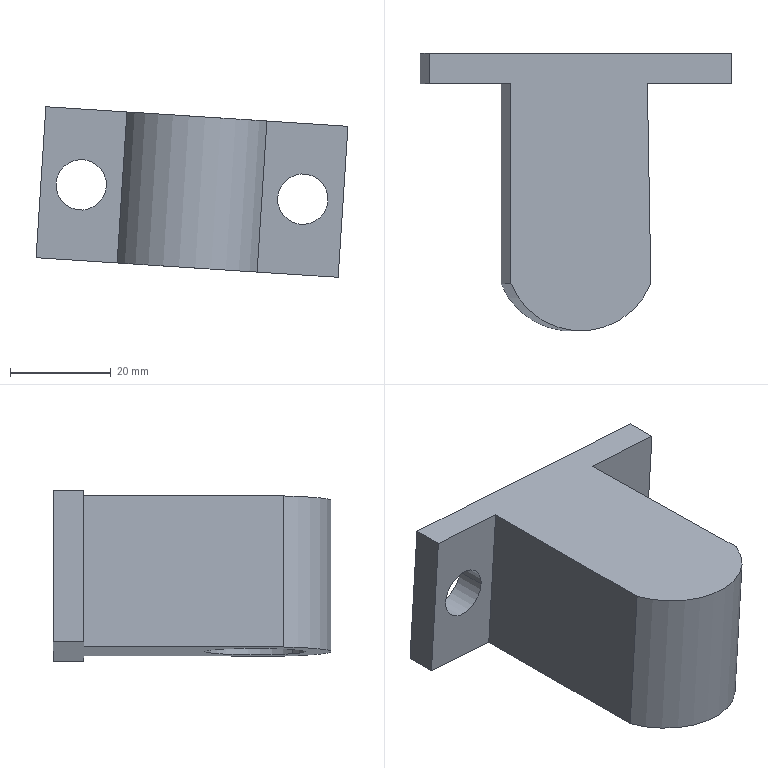Component | SolidWorks | Y-AxisBallScrewSupport2-1 | 1 solid | 17 faces | box 61.82 x 55 x 33.82 mm | volume 40291 mm3 | plane 10 | cylinder 7 | commonest cylinder face diameters 10 x4 20 x2 30 x1
build123d program:
from build123d import *

# Parameters (mm, degrees)
SKETCH1_R               = 10
BOSS_EXTRUDE1_DEPTH     = 30
SKETCH3_R               = 10
BOSS_EXTRUDE2_DEPTH     = 5
CUT_EXTRUDE1_DEPTH      = 834.997
CUT_EXTRUDE1_DEPTH_BACK = 834.997
CUT_EXTRUDE2_DEPTH      = 784.052
CUT_EXTRUDE2_DEPTH_BACK = 784.052
SKETCH5_R               = 5


with BuildPart() as part:
    # Sketch1 → Boss-Extrude1 (new body)
    with BuildSketch(Plane.XY):
        with BuildLine():
            Line((-298.984, -768.399), (-258.103, -724.481))
            Line((-258.103, -724.481), (-262.495, -720.393))
            Line((-262.495, -720.393), (-302.485, -705.168))
            ThreePointArc((-302.485, -705.168), (-318.802, -708.966), (-321.423, -725.513))
            Line((-321.423, -725.513), (-303.376, -764.311))
            Line((-303.376, -764.311), (-298.984, -768.399))
        make_face()
        with Locations((-307.822, -719.187)):
            Circle(SKETCH1_R, mode=Mode.SUBTRACT)
    extrude(amount=-BOSS_EXTRUDE1_DEPTH)

    # Sketch3 → Boss-Extrude2 (add)
    with BuildSketch(Plane.XY):
        with Locations((-307.822, -719.187)):
            Circle(SKETCH3_R)
    extrude(amount=-BOSS_EXTRUDE2_DEPTH)

    # Sketch4 → Cut-Extrude1 (cut, two sides: drawn at the far end of the back side and taken through both)
    with BuildSketch(Plane(origin=(0, 0, -30), x_dir=(-1, 0, 0), z_dir=(0, 0, -1)).offset(-CUT_EXTRUDE1_DEPTH_BACK)):
        Polygon((321.423, -725.513), (291.929, -752.014), (303.376, -764.311), align=None)
        Polygon((302.485, -705.168), (273.467, -732.18), (262.495, -720.393), align=None)
    extrude(amount=CUT_EXTRUDE1_DEPTH + CUT_EXTRUDE1_DEPTH_BACK, mode=Mode.SUBTRACT)

    # Sketch5 → Cut-Extrude2 (cut, two sides: drawn at the far end of the back side and taken through both)
    with BuildSketch(Plane(origin=(218.636, -203.516, 0), x_dir=(0, 0, 1), z_dir=(-0.732, 0.6813, 0)).offset(-CUT_EXTRUDE2_DEPTH_BACK)):
        with Locations(Location((-15, -714.151, 0), (0, 0, 90))):
            Circle(SKETCH5_R)
        with Locations(Location((-15, -758.151, 0), (0, 0, 90))):
            Circle(SKETCH5_R)
    extrude(amount=CUT_EXTRUDE2_DEPTH + CUT_EXTRUDE2_DEPTH_BACK, mode=Mode.SUBTRACT)


solid = part.part

# Placed as in the assembly
solid = solid.moved(Location((-727.162, -855.698, -137.583), (0, 3.712, 132.949)))
STEP:
#1=COLOUR_RGB('',0.7922,0.8196,0.9333);
#2=FILL_AREA_STYLE_COLOUR('',#1);
#3=FILL_AREA_STYLE('',(#2));
#4=SURFACE_STYLE_FILL_AREA(#3);
#5=SURFACE_SIDE_STYLE('',(#4));
#6=SURFACE_STYLE_USAGE(.BOTH.,#5);
#7=PRESENTATION_STYLE_ASSIGNMENT((#6));
#8=CARTESIAN_POINT('',(1.316,-21.693,-7.951));
#9=VERTEX_POINT('',#8);
#10=CARTESIAN_POINT('',(0.9228,-21.693,-7.926));
#11=VERTEX_POINT('',#10);
#12=CARTESIAN_POINT('',(1.119,-21.693,-7.938));
#13=DIRECTION('',(-0.,1.,0.));
#14=DIRECTION('',(-0.9979,0.,0.06474));
#15=AXIS2_PLACEMENT_3D('',#12,#13,#14);
#16=CIRCLE('',#15,0.1969);
#17=EDGE_CURVE('',#9,#11,#16,.T.);
#18=ORIENTED_EDGE('',*,*,#17,.T.);
#19=CARTESIAN_POINT('',(0.9228,-21.929,-7.926));
#20=VERTEX_POINT('',#19);
#21=CARTESIAN_POINT('',(0.9228,-20.515,-7.926));
#22=DIRECTION('',(-0.,-1.,0.));
#23=VECTOR('',#22,39.37);
#24=LINE('',#21,#23);
#25=EDGE_CURVE('',#11,#20,#24,.T.);
#26=ORIENTED_EDGE('',*,*,#25,.T.);
#27=CARTESIAN_POINT('',(1.316,-21.929,-7.951));
#28=VERTEX_POINT('',#27);
#29=CARTESIAN_POINT('',(1.119,-21.929,-7.938));
#30=DIRECTION('',(-0.,1.,0.));
#31=DIRECTION('',(-0.9979,0.,0.06474));
#32=AXIS2_PLACEMENT_3D('',#29,#30,#31);
#33=CIRCLE('',#32,0.1969);
#34=EDGE_CURVE('',#28,#20,#33,.T.);
#35=ORIENTED_EDGE('',*,*,#34,.F.);
#36=CARTESIAN_POINT('',(1.316,-20.515,-7.951));
#37=DIRECTION('',(-0.,-1.,0.));
#38=VECTOR('',#37,39.37);
#39=LINE('',#36,#38);
#40=EDGE_CURVE('',#9,#28,#39,.T.);
#41=ORIENTED_EDGE('',*,*,#40,.F.);
#42=EDGE_LOOP('',(#18,#26,#35,#41));
#43=FACE_OUTER_BOUND('',#42,.T.);
#44=CARTESIAN_POINT('',(1.119,-20.515,-7.938));
#45=DIRECTION('',(-0.,-1.,0.));
#46=DIRECTION('',(0.9979,0.,-0.06474));
#47=AXIS2_PLACEMENT_3D('',#44,#45,#46);
#48=CYLINDRICAL_SURFACE('',#47,0.1969);
#49=ADVANCED_FACE('',(#43),#48,.F.);
#50=CARTESIAN_POINT('',(-0.413,-21.693,-7.839));
#51=VERTEX_POINT('',#50);
#52=CARTESIAN_POINT('',(-0.8059,-21.693,-7.813));
#53=VERTEX_POINT('',#52);
#54=CARTESIAN_POINT('',(-0.6094,-21.693,-7.826));
#55=DIRECTION('',(-0.,1.,0.));
#56=DIRECTION('',(-0.9979,0.,0.06474));
#57=AXIS2_PLACEMENT_3D('',#54,#55,#56);
#58=CIRCLE('',#57,0.1969);
#59=EDGE_CURVE('',#51,#53,#58,.T.);
#60=ORIENTED_EDGE('',*,*,#59,.T.);
#61=CARTESIAN_POINT('',(-0.8059,-21.929,-7.813));
#62=VERTEX_POINT('',#61);
#63=CARTESIAN_POINT('',(-0.8059,-20.515,-7.813));
#64=DIRECTION('',(-0.,-1.,0.));
#65=VECTOR('',#64,39.37);
#66=LINE('',#63,#65);
#67=EDGE_CURVE('',#53,#62,#66,.T.);
#68=ORIENTED_EDGE('',*,*,#67,.T.);
#69=CARTESIAN_POINT('',(-0.413,-21.929,-7.839));
#70=VERTEX_POINT('',#69);
#71=CARTESIAN_POINT('',(-0.6094,-21.929,-7.826));
#72=DIRECTION('',(-0.,1.,0.));
#73=DIRECTION('',(-0.9979,0.,0.06474));
#74=AXIS2_PLACEMENT_3D('',#71,#72,#73);
#75=CIRCLE('',#74,0.1969);
#76=EDGE_CURVE('',#70,#62,#75,.T.);
#77=ORIENTED_EDGE('',*,*,#76,.F.);
#78=CARTESIAN_POINT('',(-0.413,-20.515,-7.839));
#79=DIRECTION('',(-0.,-1.,0.));
#80=VECTOR('',#79,39.37);
#81=LINE('',#78,#80);
#82=EDGE_CURVE('',#51,#70,#81,.T.);
#83=ORIENTED_EDGE('',*,*,#82,.F.);
#84=EDGE_LOOP('',(#60,#68,#77,#83));
#85=FACE_OUTER_BOUND('',#84,.T.);
#86=CARTESIAN_POINT('',(-0.6094,-20.515,-7.826));
#87=DIRECTION('',(-0.,-1.,0.));
#88=DIRECTION('',(0.9979,0.,-0.06474));
#89=AXIS2_PLACEMENT_3D('',#86,#87,#88);
#90=CYLINDRICAL_SURFACE('',#89,0.1969);
#91=ADVANCED_FACE('',(#85),#90,.F.);
#92=CARTESIAN_POINT('',(0.4843,-23.556,-8.489));
#93=VERTEX_POINT('',#92);
#94=CARTESIAN_POINT('',(-0.05103,-22.98,-8.454));
#95=VERTEX_POINT('',#94);
#96=CARTESIAN_POINT('',(0.2167,-23.268,-8.472));
#97=DIRECTION('',(0.06474,0.,0.9979));
#98=DIRECTION('',(-0.6799,0.732,0.04411));
#99=AXIS2_PLACEMENT_3D('',#96,#97,#98);
#100=CIRCLE('',#99,0.3937);
#101=EDGE_CURVE('',#93,#95,#100,.T.);
#102=ORIENTED_EDGE('',*,*,#101,.F.);
#103=CARTESIAN_POINT('',(0.5481,-23.556,-7.507));
#104=VERTEX_POINT('',#103);
#105=CARTESIAN_POINT('',(0.4843,-23.556,-8.489));
#106=DIRECTION('',(0.06474,0.,0.9979));
#107=VECTOR('',#106,39.37);
#108=LINE('',#105,#107);
#109=EDGE_CURVE('',#93,#104,#108,.T.);
#110=ORIENTED_EDGE('',*,*,#109,.T.);
#111=CARTESIAN_POINT('',(0.01269,-22.98,-7.472));
#112=VERTEX_POINT('',#111);
#113=CARTESIAN_POINT('',(0.2804,-23.268,-7.489));
#114=DIRECTION('',(-0.06474,-0.,-0.9979));
#115=DIRECTION('',(-0.6799,0.732,0.04411));
#116=AXIS2_PLACEMENT_3D('',#113,#114,#115);
#117=CIRCLE('',#116,0.3937);
#118=EDGE_CURVE('',#112,#104,#117,.T.);
#119=ORIENTED_EDGE('',*,*,#118,.F.);
#120=CARTESIAN_POINT('',(-0.05103,-22.98,-8.454));
#121=DIRECTION('',(0.06474,0.,0.9979));
#122=VECTOR('',#121,39.37);
#123=LINE('',#120,#122);
#124=EDGE_CURVE('',#95,#112,#123,.T.);
#125=ORIENTED_EDGE('',*,*,#124,.F.);
#126=EDGE_LOOP('',(#102,#110,#119,#125));
#127=FACE_OUTER_BOUND('',#126,.T.);
#128=CARTESIAN_POINT('',(0.2167,-23.268,-8.472));
#129=DIRECTION('',(0.06474,0.,0.9979));
#130=DIRECTION('',(-0.6799,0.732,0.04411));
#131=AXIS2_PLACEMENT_3D('',#128,#129,#130);
#132=CYLINDRICAL_SURFACE('',#131,0.3937);
#133=ADVANCED_FACE('',(#127),#132,.F.);
#134=ORIENTED_EDGE('',*,*,#109,.F.);
#135=CARTESIAN_POINT('',(0.2167,-23.268,-8.472));
#136=DIRECTION('',(0.06474,0.,0.9979));
#137=DIRECTION('',(-0.6799,0.732,0.04411));
#138=AXIS2_PLACEMENT_3D('',#135,#136,#137);
#139=CIRCLE('',#138,0.3937);
#140=EDGE_CURVE('',#95,#93,#139,.T.);
#141=ORIENTED_EDGE('',*,*,#140,.F.);
#142=ORIENTED_EDGE('',*,*,#124,.T.);
#143=CARTESIAN_POINT('',(0.2804,-23.268,-7.489));
#144=DIRECTION('',(-0.06474,-0.,-0.9979));
#145=DIRECTION('',(-0.6799,0.732,0.04411));
#146=AXIS2_PLACEMENT_3D('',#143,#144,#145);
#147=CIRCLE('',#146,0.3937);
#148=EDGE_CURVE('',#104,#112,#147,.T.);
#149=ORIENTED_EDGE('',*,*,#148,.F.);
#150=EDGE_LOOP('',(#134,#141,#142,#149));
#151=FACE_OUTER_BOUND('',#150,.T.);
#152=CARTESIAN_POINT('',(0.2167,-23.268,-8.472));
#153=DIRECTION('',(0.06474,0.,0.9979));
#154=DIRECTION('',(-0.6799,0.732,0.04411));
#155=AXIS2_PLACEMENT_3D('',#152,#153,#154);
#156=CYLINDRICAL_SURFACE('',#155,0.3937);
#157=ADVANCED_FACE('',(#151),#156,.F.);
#158=CARTESIAN_POINT('',(1.472,-21.693,-7.369));
#159=VERTEX_POINT('',#158);
#160=CARTESIAN_POINT('',(1.472,-21.929,-7.369));
#161=VERTEX_POINT('',#160);
#162=CARTESIAN_POINT('',(1.472,-33.689,-7.369));
#163=DIRECTION('',(0.,-1.,-0.));
#164=VECTOR('',#163,39.37);
#165=LINE('',#162,#164);
#166=EDGE_CURVE('',#159,#161,#165,.T.);
#167=ORIENTED_EDGE('',*,*,#166,.T.);
#168=CARTESIAN_POINT('',(1.395,-21.929,-8.548));
#169=VERTEX_POINT('',#168);
#170=CARTESIAN_POINT('',(1.395,-21.929,-8.548));
#171=DIRECTION('',(0.06474,0.,0.9979));
#172=VECTOR('',#171,39.37);
#173=LINE('',#170,#172);
#174=EDGE_CURVE('',#169,#161,#173,.T.);
#175=ORIENTED_EDGE('',*,*,#174,.F.);
#176=CARTESIAN_POINT('',(1.395,-21.693,-8.548));
#177=VERTEX_POINT('',#176);
#178=CARTESIAN_POINT('',(1.395,-33.689,-8.548));
#179=DIRECTION('',(0.,-1.,-0.));
#180=VECTOR('',#179,39.37);
#181=LINE('',#178,#180);
#182=EDGE_CURVE('',#177,#169,#181,.T.);
#183=ORIENTED_EDGE('',*,*,#182,.F.);
#184=CARTESIAN_POINT('',(1.395,-21.693,-8.548));
#185=DIRECTION('',(0.06474,0.,0.9979));
#186=VECTOR('',#185,39.37);
#187=LINE('',#184,#186);
#188=EDGE_CURVE('',#177,#159,#187,.T.);
#189=ORIENTED_EDGE('',*,*,#188,.T.);
#190=EDGE_LOOP('',(#167,#175,#183,#189));
#191=FACE_OUTER_BOUND('',#190,.T.);
#192=CARTESIAN_POINT('',(1.395,-33.689,-8.548));
#193=DIRECTION('',(-0.9979,-0.,0.06474));
#194=DIRECTION('',(0.,-1.,-0.));
#195=AXIS2_PLACEMENT_3D('',#192,#193,#194);
#196=PLANE('',#195);
#197=ADVANCED_FACE('',(#191),#196,.F.);
#198=CARTESIAN_POINT('',(-0.2529,-23.49,-7.258));
#199=VERTEX_POINT('',#198);
#200=CARTESIAN_POINT('',(0.8391,-23.49,-7.328));
#201=VERTEX_POINT('',#200);
#202=CARTESIAN_POINT('',(0.2931,-23.268,-7.293));
#203=DIRECTION('',(0.06474,0.,0.9979));
#204=DIRECTION('',(-0.6799,0.732,0.04411));
#205=AXIS2_PLACEMENT_3D('',#202,#203,#204);
#206=CIRCLE('',#205,0.5906);
#207=EDGE_CURVE('',#199,#201,#206,.T.);
#208=ORIENTED_EDGE('',*,*,#207,.F.);
#209=CARTESIAN_POINT('',(-0.3293,-23.49,-8.436));
#210=VERTEX_POINT('',#209);
#211=CARTESIAN_POINT('',(-0.3293,-23.49,-8.436));
#212=DIRECTION('',(0.06474,0.,0.9979));
#213=VECTOR('',#212,39.37);
#214=LINE('',#211,#213);
#215=EDGE_CURVE('',#210,#199,#214,.T.);
#216=ORIENTED_EDGE('',*,*,#215,.F.);
#217=CARTESIAN_POINT('',(0.7626,-23.49,-8.507));
#218=VERTEX_POINT('',#217);
#219=CARTESIAN_POINT('',(0.2167,-23.268,-8.472));
#220=DIRECTION('',(0.06474,0.,0.9979));
#221=DIRECTION('',(-0.6799,0.732,0.04411));
#222=AXIS2_PLACEMENT_3D('',#219,#220,#221);
#223=CIRCLE('',#222,0.5906);
#224=EDGE_CURVE('',#210,#218,#223,.T.);
#225=ORIENTED_EDGE('',*,*,#224,.T.);
#226=CARTESIAN_POINT('',(0.7626,-23.49,-8.507));
#227=DIRECTION('',(0.06474,0.,0.9979));
#228=VECTOR('',#227,39.37);
#229=LINE('',#226,#228);
#230=EDGE_CURVE('',#218,#201,#229,.T.);
#231=ORIENTED_EDGE('',*,*,#230,.T.);
#232=EDGE_LOOP('',(#208,#216,#225,#231));
#233=FACE_OUTER_BOUND('',#232,.T.);
#234=CARTESIAN_POINT('',(0.2167,-23.268,-8.472));
#235=DIRECTION('',(0.06474,0.,0.9979));
#236=DIRECTION('',(-0.6799,0.732,0.04411));
#237=AXIS2_PLACEMENT_3D('',#234,#235,#236);
#238=CYLINDRICAL_SURFACE('',#237,0.5906);
#239=ADVANCED_FACE('',(#233),#238,.T.);
#240=CARTESIAN_POINT('',(-0.8855,-21.693,-7.216));
#241=VERTEX_POINT('',#240);
#242=CARTESIAN_POINT('',(-0.8855,-21.929,-7.216));
#243=VERTEX_POINT('',#242);
#244=CARTESIAN_POINT('',(-0.8855,-33.689,-7.216));
#245=DIRECTION('',(-0.,-1.,0.));
#246=VECTOR('',#245,39.37);
#247=LINE('',#244,#246);
#248=EDGE_CURVE('',#241,#243,#247,.T.);
#249=ORIENTED_EDGE('',*,*,#248,.F.);
#250=CARTESIAN_POINT('',(-0.962,-21.693,-8.395));
#251=VERTEX_POINT('',#250);
#252=CARTESIAN_POINT('',(-0.962,-21.693,-8.395));
#253=DIRECTION('',(0.06474,0.,0.9979));
#254=VECTOR('',#253,39.37);
#255=LINE('',#252,#254);
#256=EDGE_CURVE('',#251,#241,#255,.T.);
#257=ORIENTED_EDGE('',*,*,#256,.F.);
#258=CARTESIAN_POINT('',(-0.962,-21.929,-8.395));
#259=VERTEX_POINT('',#258);
#260=CARTESIAN_POINT('',(-0.962,-33.689,-8.395));
#261=DIRECTION('',(-0.,-1.,0.));
#262=VECTOR('',#261,39.37);
#263=LINE('',#260,#262);
#264=EDGE_CURVE('',#251,#259,#263,.T.);
#265=ORIENTED_EDGE('',*,*,#264,.T.);
#266=CARTESIAN_POINT('',(-0.962,-21.929,-8.395));
#267=DIRECTION('',(0.06474,0.,0.9979));
#268=VECTOR('',#267,39.37);
#269=LINE('',#266,#268);
#270=EDGE_CURVE('',#259,#243,#269,.T.);
#271=ORIENTED_EDGE('',*,*,#270,.T.);
#272=EDGE_LOOP('',(#249,#257,#265,#271));
#273=FACE_OUTER_BOUND('',#272,.T.);
#274=CARTESIAN_POINT('',(-0.962,-33.689,-8.395));
#275=DIRECTION('',(-0.9979,0.,0.06474));
#276=DIRECTION('',(-0.,-1.,0.));
#277=AXIS2_PLACEMENT_3D('',#274,#275,#276);
#278=PLANE('',#277);
#279=ADVANCED_FACE('',(#273),#278,.T.);
#280=ORIENTED_EDGE('',*,*,#17,.F.);
#281=CARTESIAN_POINT('',(1.119,-21.693,-7.938));
#282=DIRECTION('',(-0.,1.,0.));
#283=DIRECTION('',(-0.9979,0.,0.06474));
#284=AXIS2_PLACEMENT_3D('',#281,#282,#283);
#285=CIRCLE('',#284,0.1969);
#286=EDGE_CURVE('',#11,#9,#285,.T.);
#287=ORIENTED_EDGE('',*,*,#286,.F.);
#288=EDGE_LOOP('',(#280,#287));
#289=FACE_BOUND('',#288,.T.);
#290=ORIENTED_EDGE('',*,*,#59,.F.);
#291=CARTESIAN_POINT('',(-0.6094,-21.693,-7.826));
#292=DIRECTION('',(-0.,1.,0.));
#293=DIRECTION('',(-0.9979,0.,0.06474));
#294=AXIS2_PLACEMENT_3D('',#291,#292,#293);
#295=CIRCLE('',#294,0.1969);
#296=EDGE_CURVE('',#53,#51,#295,.T.);
#297=ORIENTED_EDGE('',*,*,#296,.F.);
#298=EDGE_LOOP('',(#290,#297));
#299=FACE_BOUND('',#298,.T.);
#300=CARTESIAN_POINT('',(-28.628,-21.693,-5.417));
#301=DIRECTION('',(-0.9979,-0.,0.06474));
#302=VECTOR('',#301,39.37);
#303=LINE('',#300,#302);
#304=EDGE_CURVE('',#159,#241,#303,.T.);
#305=ORIENTED_EDGE('',*,*,#304,.F.);
#306=ORIENTED_EDGE('',*,*,#188,.F.);
#307=CARTESIAN_POINT('',(-28.705,-21.693,-6.595));
#308=DIRECTION('',(-0.9979,-0.,0.06474));
#309=VECTOR('',#308,39.37);
#310=LINE('',#307,#309);
#311=EDGE_CURVE('',#177,#251,#310,.T.);
#312=ORIENTED_EDGE('',*,*,#311,.T.);
#313=ORIENTED_EDGE('',*,*,#256,.T.);
#314=EDGE_LOOP('',(#305,#306,#312,#313));
#315=FACE_OUTER_BOUND('',#314,.T.);
#316=CARTESIAN_POINT('',(-28.705,-21.693,-6.595));
#317=DIRECTION('',(-0.,1.,0.));
#318=DIRECTION('',(-0.9979,-0.,0.06474));
#319=AXIS2_PLACEMENT_3D('',#316,#317,#318);
#320=PLANE('',#319);
#321=ADVANCED_FACE('',(#289,#299,#315),#320,.T.);
#322=CARTESIAN_POINT('',(-0.3293,-21.929,-8.436));
#323=VERTEX_POINT('',#322);
#324=CARTESIAN_POINT('',(-0.3293,-33.689,-8.436));
#325=DIRECTION('',(0.,1.,-0.));
#326=VECTOR('',#325,39.37);
#327=LINE('',#324,#326);
#328=EDGE_CURVE('',#210,#323,#327,.T.);
#329=ORIENTED_EDGE('',*,*,#328,.T.);
#330=CARTESIAN_POINT('',(-28.705,-21.929,-6.595));
#331=DIRECTION('',(-0.9979,-0.,0.06474));
#332=VECTOR('',#331,39.37);
#333=LINE('',#330,#332);
#334=EDGE_CURVE('',#323,#259,#333,.T.);
#335=ORIENTED_EDGE('',*,*,#334,.T.);
#336=ORIENTED_EDGE('',*,*,#264,.F.);
#337=ORIENTED_EDGE('',*,*,#311,.F.);
#338=ORIENTED_EDGE('',*,*,#182,.T.);
#339=CARTESIAN_POINT('',(0.7352,-21.929,-8.505));
#340=VERTEX_POINT('',#339);
#341=CARTESIAN_POINT('',(-28.705,-21.929,-6.595));
#342=DIRECTION('',(-0.9979,-0.,0.06474));
#343=VECTOR('',#342,39.37);
#344=LINE('',#341,#343);
#345=EDGE_CURVE('',#169,#340,#344,.T.);
#346=ORIENTED_EDGE('',*,*,#345,.T.);
#347=CARTESIAN_POINT('',(0.9325,-33.166,-8.518));
#348=DIRECTION('',(0.01755,-0.9998,-0.001139));
#349=VECTOR('',#348,39.37);
#350=LINE('',#347,#349);
#351=EDGE_CURVE('',#340,#218,#350,.T.);
#352=ORIENTED_EDGE('',*,*,#351,.T.);
#353=ORIENTED_EDGE('',*,*,#224,.F.);
#354=EDGE_LOOP('',(#329,#335,#336,#337,#338,#346,#352,#353));
#355=FACE_OUTER_BOUND('',#354,.T.);
#356=ORIENTED_EDGE('',*,*,#140,.T.);
#357=ORIENTED_EDGE('',*,*,#101,.T.);
#358=EDGE_LOOP('',(#356,#357));
#359=FACE_BOUND('',#358,.T.);
#360=CARTESIAN_POINT('',(-28.705,-33.689,-6.595));
#361=DIRECTION('',(0.06474,-0.,0.9979));
#362=DIRECTION('',(-0.6799,0.732,0.04411));
#363=AXIS2_PLACEMENT_3D('',#360,#361,#362);
#364=PLANE('',#363);
#365=ADVANCED_FACE('',(#355,#359),#364,.F.);
#366=CARTESIAN_POINT('',(-0.2529,-21.929,-7.258));
#367=VERTEX_POINT('',#366);
#368=CARTESIAN_POINT('',(-0.8855,-21.929,-7.216));
#369=DIRECTION('',(0.9979,0.,-0.06474));
#370=VECTOR('',#369,39.37);
#371=LINE('',#368,#370);
#372=EDGE_CURVE('',#243,#367,#371,.T.);
#373=ORIENTED_EDGE('',*,*,#372,.T.);
#374=CARTESIAN_POINT('',(-0.2529,-23.49,-7.258));
#375=DIRECTION('',(-0.,-1.,0.));
#376=VECTOR('',#375,39.37);
#377=LINE('',#374,#376);
#378=EDGE_CURVE('',#367,#199,#377,.T.);
#379=ORIENTED_EDGE('',*,*,#378,.T.);
#380=ORIENTED_EDGE('',*,*,#207,.T.);
#381=CARTESIAN_POINT('',(0.8117,-21.929,-7.327));
#382=VERTEX_POINT('',#381);
#383=CARTESIAN_POINT('',(0.8391,-23.49,-7.328));
#384=DIRECTION('',(-0.01755,0.9998,0.001139));
#385=VECTOR('',#384,39.37);
#386=LINE('',#383,#385);
#387=EDGE_CURVE('',#201,#382,#386,.T.);
#388=ORIENTED_EDGE('',*,*,#387,.T.);
#389=CARTESIAN_POINT('',(0.8117,-21.929,-7.327));
#390=DIRECTION('',(0.9979,0.,-0.06474));
#391=VECTOR('',#390,39.37);
#392=LINE('',#389,#391);
#393=EDGE_CURVE('',#382,#161,#392,.T.);
#394=ORIENTED_EDGE('',*,*,#393,.T.);
#395=ORIENTED_EDGE('',*,*,#166,.F.);
#396=ORIENTED_EDGE('',*,*,#304,.T.);
#397=ORIENTED_EDGE('',*,*,#248,.T.);
#398=EDGE_LOOP('',(#373,#379,#380,#388,#394,#395,#396,#397));
#399=FACE_OUTER_BOUND('',#398,.T.);
#400=CARTESIAN_POINT('',(-28.628,-33.689,-5.417));
#401=DIRECTION('',(0.06474,-0.,0.9979));
#402=DIRECTION('',(-0.6799,0.732,0.04411));
#403=AXIS2_PLACEMENT_3D('',#400,#401,#402);
#404=PLANE('',#403);
#405=ADVANCED_FACE('',(#399),#404,.T.);
#406=ORIENTED_EDGE('',*,*,#118,.T.);
#407=ORIENTED_EDGE('',*,*,#148,.T.);
#408=EDGE_LOOP('',(#406,#407));
#409=FACE_OUTER_BOUND('',#408,.T.);
#410=CARTESIAN_POINT('',(0.2804,-23.268,-7.489));
#411=DIRECTION('',(0.06474,-0.,0.9979));
#412=DIRECTION('',(-0.6799,0.732,0.04411));
#413=AXIS2_PLACEMENT_3D('',#410,#411,#412);
#414=PLANE('',#413);
#415=ADVANCED_FACE('',(#409),#414,.F.);
#416=ORIENTED_EDGE('',*,*,#34,.T.);
#417=CARTESIAN_POINT('',(1.119,-21.929,-7.938));
#418=DIRECTION('',(-0.,1.,0.));
#419=DIRECTION('',(-0.9979,0.,0.06474));
#420=AXIS2_PLACEMENT_3D('',#417,#418,#419);
#421=CIRCLE('',#420,0.1969);
#422=EDGE_CURVE('',#20,#28,#421,.T.);
#423=ORIENTED_EDGE('',*,*,#422,.T.);
#424=EDGE_LOOP('',(#416,#423));
#425=FACE_BOUND('',#424,.T.);
#426=ORIENTED_EDGE('',*,*,#174,.T.);
#427=ORIENTED_EDGE('',*,*,#393,.F.);
#428=CARTESIAN_POINT('',(0.8117,-21.929,-7.327));
#429=DIRECTION('',(-0.06474,-0.,-0.9979));
#430=VECTOR('',#429,39.37);
#431=LINE('',#428,#430);
#432=EDGE_CURVE('',#382,#340,#431,.T.);
#433=ORIENTED_EDGE('',*,*,#432,.T.);
#434=ORIENTED_EDGE('',*,*,#345,.F.);
#435=EDGE_LOOP('',(#426,#427,#433,#434));
#436=FACE_OUTER_BOUND('',#435,.T.);
#437=CARTESIAN_POINT('',(0.8117,-21.929,-7.327));
#438=DIRECTION('',(-0.,1.,0.));
#439=DIRECTION('',(-0.9979,-0.,0.06474));
#440=AXIS2_PLACEMENT_3D('',#437,#438,#439);
#441=PLANE('',#440);
#442=ADVANCED_FACE('',(#425,#436),#441,.F.);
#443=ORIENTED_EDGE('',*,*,#432,.F.);
#444=ORIENTED_EDGE('',*,*,#387,.F.);
#445=ORIENTED_EDGE('',*,*,#230,.F.);
#446=ORIENTED_EDGE('',*,*,#351,.F.);
#447=EDGE_LOOP('',(#443,#444,#445,#446));
#448=FACE_OUTER_BOUND('',#447,.T.);
#449=CARTESIAN_POINT('',(0.8391,-23.49,-7.328));
#450=DIRECTION('',(-0.9977,-0.01759,0.06473));
#451=DIRECTION('',(0.01755,-0.9998,-0.001139));
#452=AXIS2_PLACEMENT_3D('',#449,#450,#451);
#453=PLANE('',#452);
#454=ADVANCED_FACE('',(#448),#453,.F.);
#455=ORIENTED_EDGE('',*,*,#76,.T.);
#456=CARTESIAN_POINT('',(-0.6094,-21.929,-7.826));
#457=DIRECTION('',(-0.,1.,0.));
#458=DIRECTION('',(-0.9979,0.,0.06474));
#459=AXIS2_PLACEMENT_3D('',#456,#457,#458);
#460=CIRCLE('',#459,0.1969);
#461=EDGE_CURVE('',#62,#70,#460,.T.);
#462=ORIENTED_EDGE('',*,*,#461,.T.);
#463=EDGE_LOOP('',(#455,#462));
#464=FACE_BOUND('',#463,.T.);
#465=CARTESIAN_POINT('',(-0.2529,-21.929,-7.258));
#466=DIRECTION('',(-0.06474,-0.,-0.9979));
#467=VECTOR('',#466,39.37);
#468=LINE('',#465,#467);
#469=EDGE_CURVE('',#367,#323,#468,.T.);
#470=ORIENTED_EDGE('',*,*,#469,.F.);
#471=ORIENTED_EDGE('',*,*,#372,.F.);
#472=ORIENTED_EDGE('',*,*,#270,.F.);
#473=ORIENTED_EDGE('',*,*,#334,.F.);
#474=EDGE_LOOP('',(#470,#471,#472,#473));
#475=FACE_OUTER_BOUND('',#474,.T.);
#476=CARTESIAN_POINT('',(-0.8855,-21.929,-7.216));
#477=DIRECTION('',(-0.,1.,0.));
#478=DIRECTION('',(-0.9979,-0.,0.06474));
#479=AXIS2_PLACEMENT_3D('',#476,#477,#478);
#480=PLANE('',#479);
#481=ADVANCED_FACE('',(#464,#475),#480,.F.);
#482=ORIENTED_EDGE('',*,*,#215,.T.);
#483=ORIENTED_EDGE('',*,*,#378,.F.);
#484=ORIENTED_EDGE('',*,*,#469,.T.);
#485=ORIENTED_EDGE('',*,*,#328,.F.);
#486=EDGE_LOOP('',(#482,#483,#484,#485));
#487=FACE_OUTER_BOUND('',#486,.T.);
#488=CARTESIAN_POINT('',(-0.2529,-23.49,-7.258));
#489=DIRECTION('',(0.9979,-0.,-0.06474));
#490=DIRECTION('',(0.,1.,-0.));
#491=AXIS2_PLACEMENT_3D('',#488,#489,#490);
#492=PLANE('',#491);
#493=ADVANCED_FACE('',(#487),#492,.F.);
#494=ORIENTED_EDGE('',*,*,#67,.F.);
#495=ORIENTED_EDGE('',*,*,#296,.T.);
#496=ORIENTED_EDGE('',*,*,#82,.T.);
#497=ORIENTED_EDGE('',*,*,#461,.F.);
#498=EDGE_LOOP('',(#494,#495,#496,#497));
#499=FACE_OUTER_BOUND('',#498,.T.);
#500=CARTESIAN_POINT('',(-0.6094,-20.515,-7.826));
#501=DIRECTION('',(-0.,-1.,0.));
#502=DIRECTION('',(0.9979,0.,-0.06474));
#503=AXIS2_PLACEMENT_3D('',#500,#501,#502);
#504=CYLINDRICAL_SURFACE('',#503,0.1969);
#505=ADVANCED_FACE('',(#499),#504,.F.);
#506=ORIENTED_EDGE('',*,*,#25,.F.);
#507=ORIENTED_EDGE('',*,*,#286,.T.);
#508=ORIENTED_EDGE('',*,*,#40,.T.);
#509=ORIENTED_EDGE('',*,*,#422,.F.);
#510=EDGE_LOOP('',(#506,#507,#508,#509));
#511=FACE_OUTER_BOUND('',#510,.T.);
#512=CARTESIAN_POINT('',(1.119,-20.515,-7.938));
#513=DIRECTION('',(-0.,-1.,0.));
#514=DIRECTION('',(0.9979,0.,-0.06474));
#515=AXIS2_PLACEMENT_3D('',#512,#513,#514);
#516=CYLINDRICAL_SURFACE('',#515,0.1969);
#517=ADVANCED_FACE('',(#511),#516,.F.);
#518=CLOSED_SHELL('',(#49,#91,#133,#157,#197,#239,#279,#321,#365,#405,#415,#442,#454,#481,#493,#505,#517));
#519=MANIFOLD_SOLID_BREP('',#518);
#520=STYLED_ITEM('',(#7),#519);
#521=PRESENTATION_LAYER_ASSIGNMENT('','',(#520));
#522=(LENGTH_UNIT()NAMED_UNIT(*)SI_UNIT($,.METRE.));
#523=LENGTH_MEASURE_WITH_UNIT(LENGTH_MEASURE(0.0254),#522);
#524=DIMENSIONAL_EXPONENTS(1.,0.,0.,0.,0.,0.,0.);
#525=(CONVERSION_BASED_UNIT('',#523)LENGTH_UNIT()NAMED_UNIT(#524));
#526=UNCERTAINTY_MEASURE_WITH_UNIT(LENGTH_MEASURE(0.00001),#525,'','');
#527=(NAMED_UNIT(*)PLANE_ANGLE_UNIT()SI_UNIT($,.RADIAN.));
#528=(NAMED_UNIT(*)SI_UNIT($,.STERADIAN.)SOLID_ANGLE_UNIT());
#529=(GEOMETRIC_REPRESENTATION_CONTEXT(3)GLOBAL_UNCERTAINTY_ASSIGNED_CONTEXT((#526))GLOBAL_UNIT_ASSIGNED_CONTEXT((#525,#527,#528))REPRESENTATION_CONTEXT('',''));
#530=MECHANICAL_DESIGN_GEOMETRIC_PRESENTATION_REPRESENTATION('',(#520),#529);
#531=CARTESIAN_POINT('',(0.,0.,0.));
#532=DIRECTION('',(0.,0.,1.));
#533=DIRECTION('',(1.,0.,0.));
#534=AXIS2_PLACEMENT_3D('',#531,#532,#533);
#535=(LENGTH_UNIT()NAMED_UNIT(*)SI_UNIT($,.METRE.));
#536=LENGTH_MEASURE_WITH_UNIT(LENGTH_MEASURE(0.0254),#535);
#537=DIMENSIONAL_EXPONENTS(1.,0.,0.,0.,0.,0.,0.);
#538=(CONVERSION_BASED_UNIT('',#536)LENGTH_UNIT()NAMED_UNIT(#537));
#539=UNCERTAINTY_MEASURE_WITH_UNIT(LENGTH_MEASURE(0.00001),#538,'','');
#540=(NAMED_UNIT(*)PLANE_ANGLE_UNIT()SI_UNIT($,.RADIAN.));
#541=(NAMED_UNIT(*)SI_UNIT($,.STERADIAN.)SOLID_ANGLE_UNIT());
#542=(GEOMETRIC_REPRESENTATION_CONTEXT(3)GLOBAL_UNCERTAINTY_ASSIGNED_CONTEXT((#539))GLOBAL_UNIT_ASSIGNED_CONTEXT((#538,#540,#541))REPRESENTATION_CONTEXT('',''));
#543=ADVANCED_BREP_SHAPE_REPRESENTATION('',(#519,#534),#542);